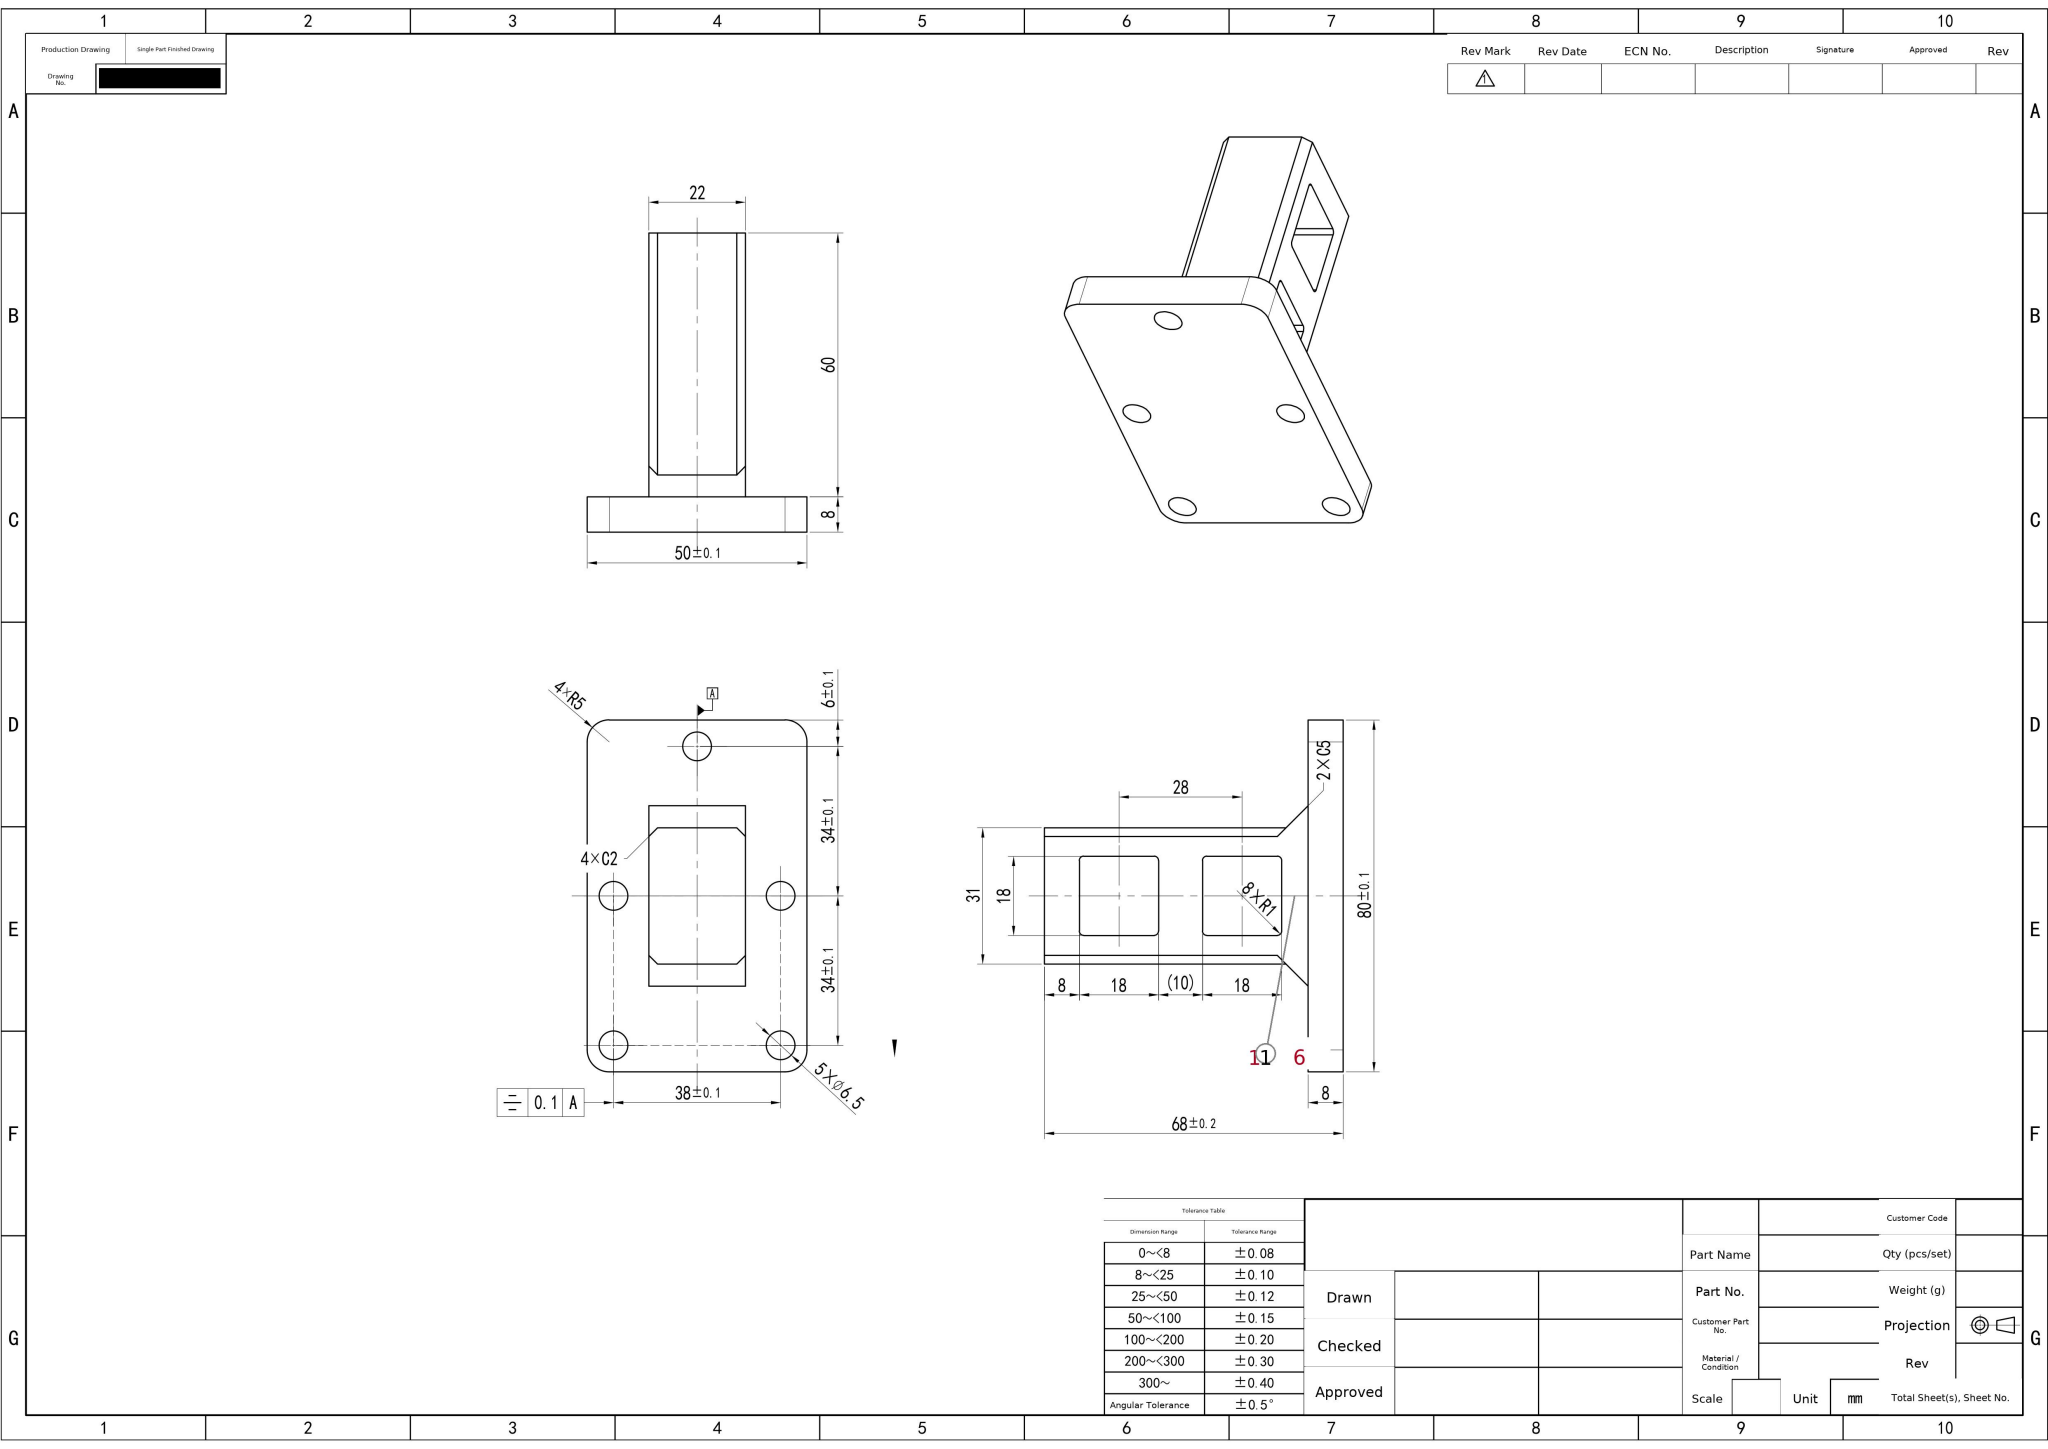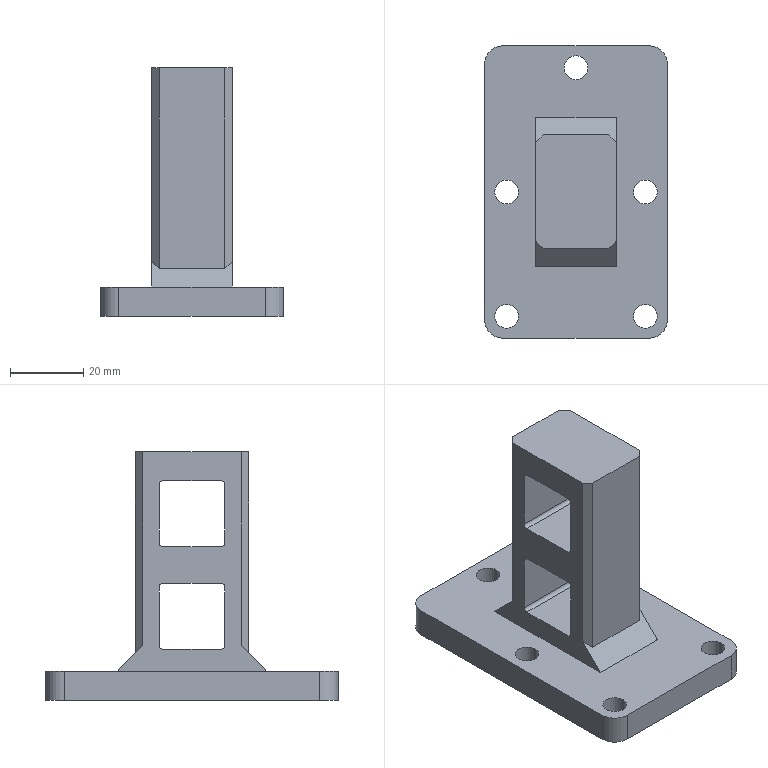Part | SolidWorks | mm | 1 solid | 47 faces | box 50 x 80 x 68 mm | volume 57318 mm3 | plane 25 | cylinder 22 | commonest cylinder face diameters 6.5 x10 2 x8 10 x4